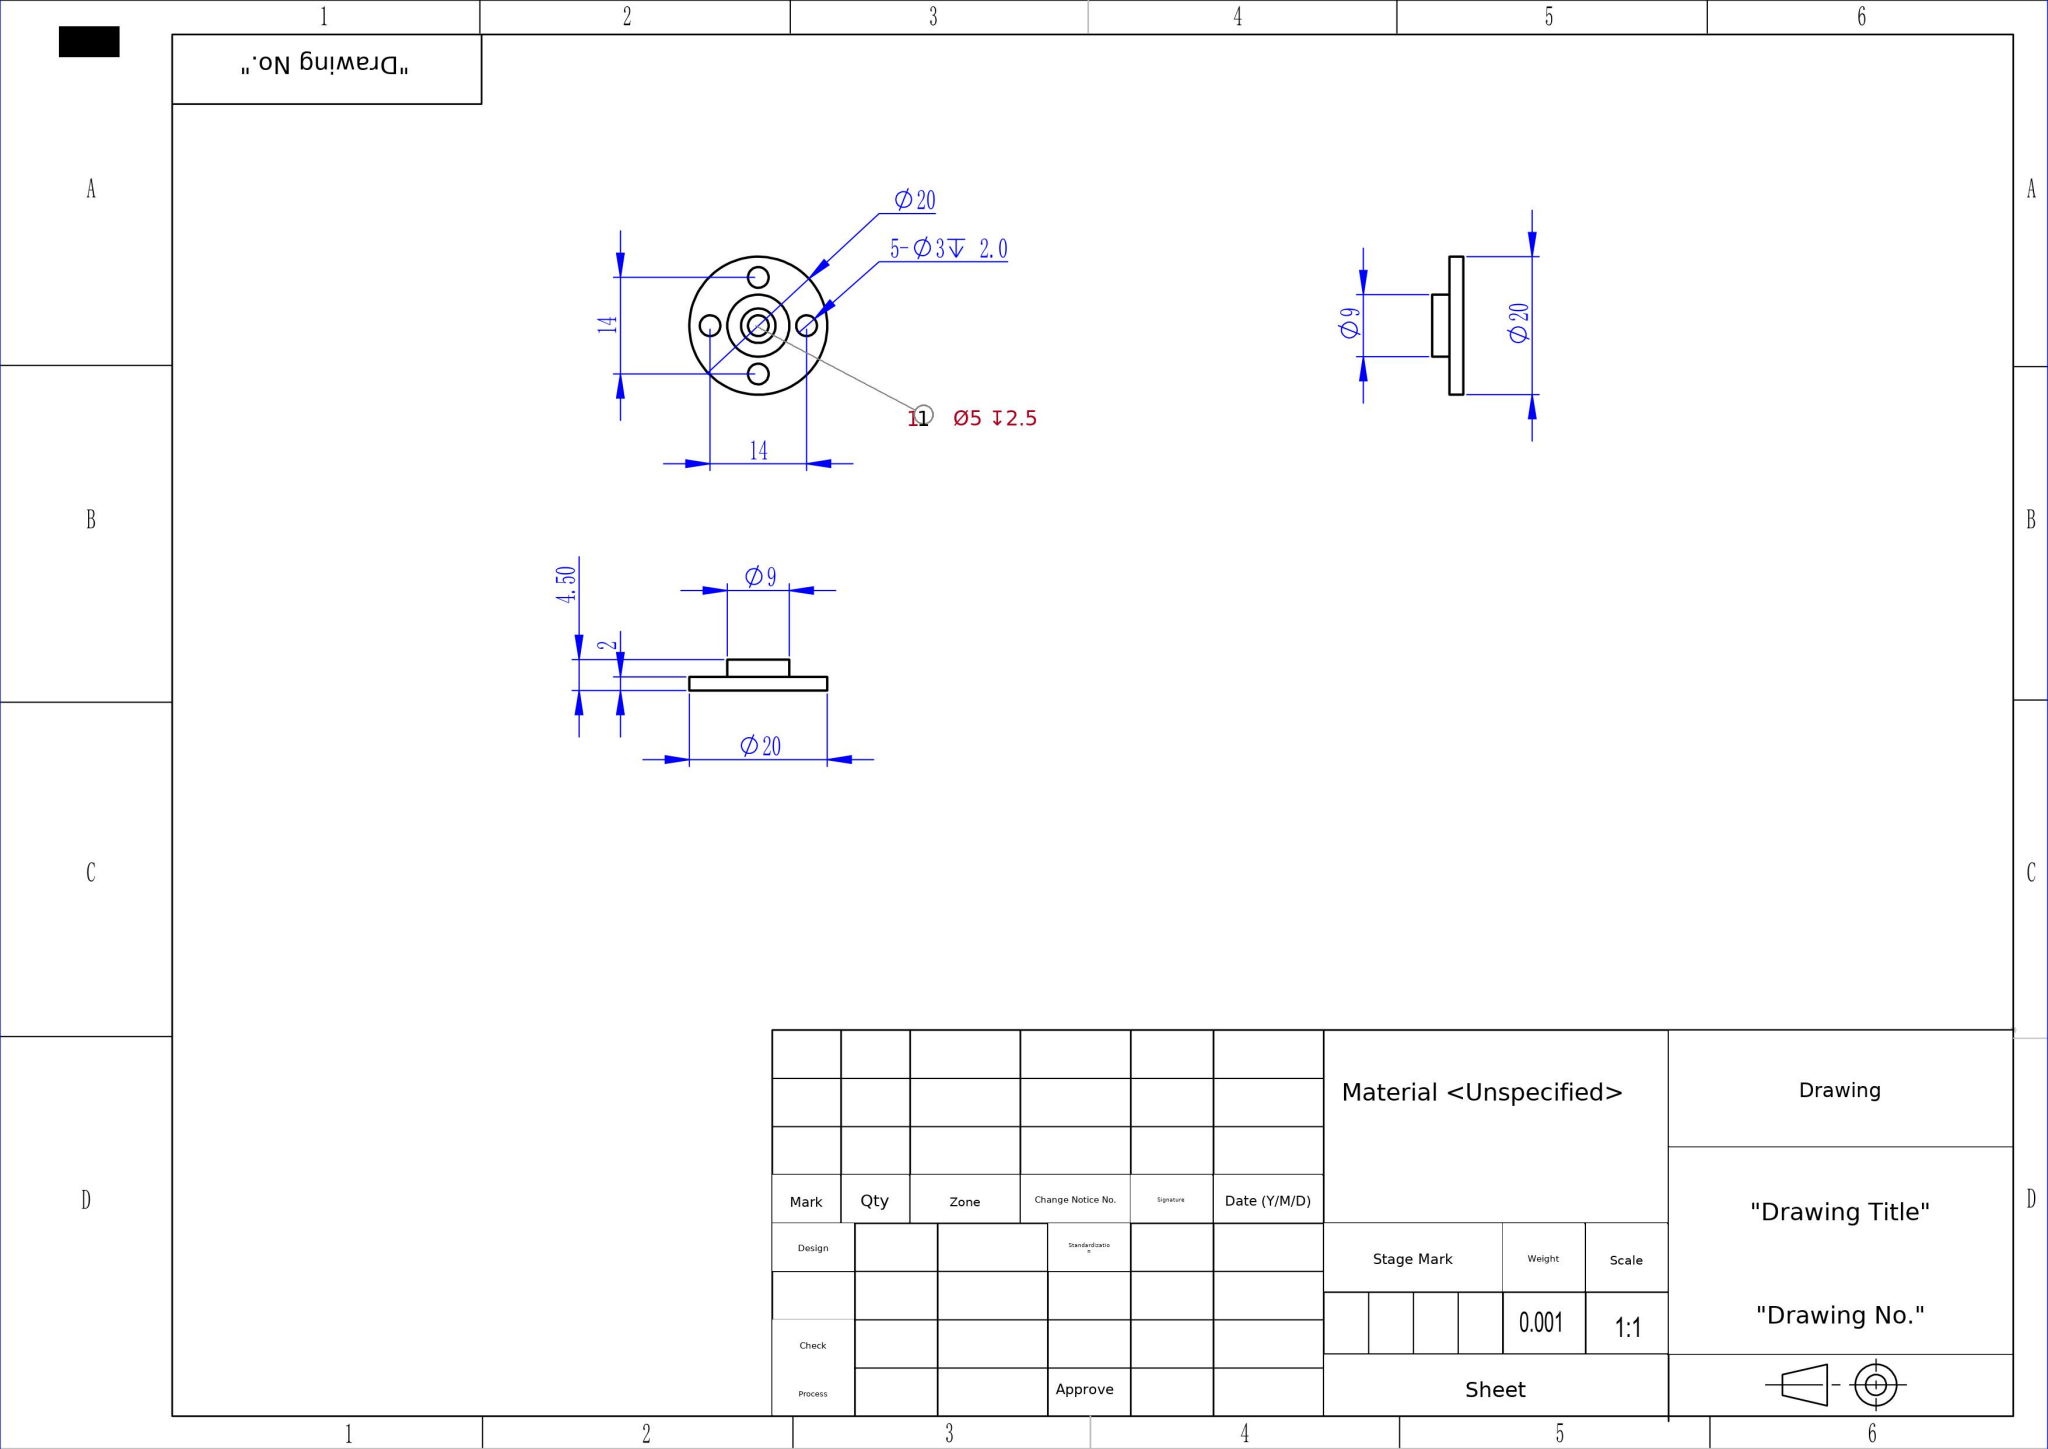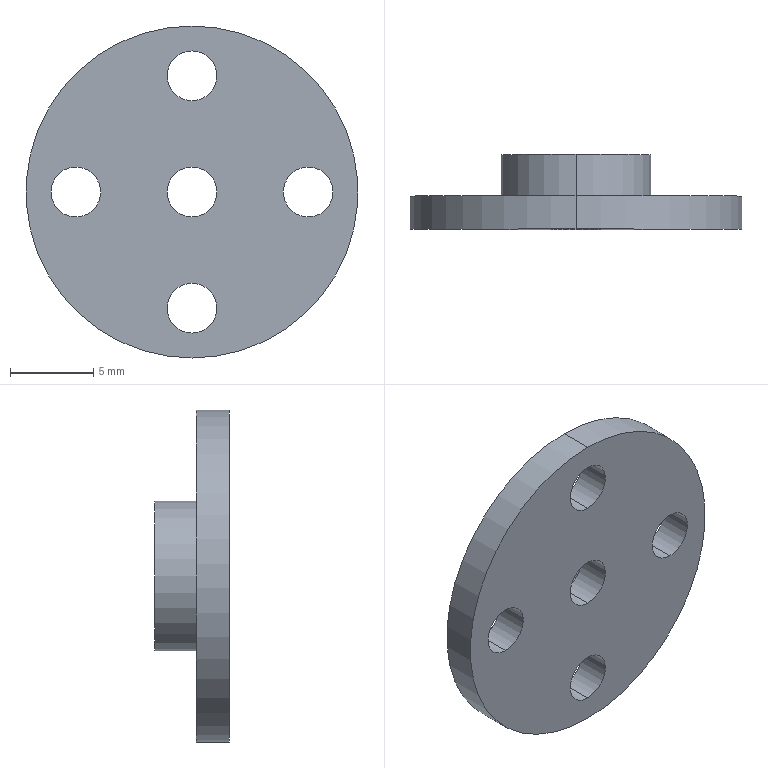Part | SolidWorks | mm | 1 solid | 20 faces | box 20 x 4.5 x 20 mm | volume 668 mm3 | cylinder 16 | plane 4 | commonest cylinder face diameters 3 x10 5 x2 9 x2 20 x2
build123d program:
from build123d import *

# Parameters (mm, degrees)
SKETCH1_R           = 10
BOSS_EXTRUDE1_DEPTH = 2
SKETCH2_R           = 1.5
CUT_EXTRUDE1_DEPTH  = 2
SKETCH3_R           = 4.5
SKETCH3_R_2         = 2.5
BOSS_EXTRUDE2_DEPTH = 2.5


with BuildPart() as part:
    # Sketch1 → Boss-Extrude1 (new body)
    with BuildSketch(Plane(origin=(0, 0, 0), x_dir=(1, 0, 0), z_dir=(0, 1, 0))):
        with Locations(Location((0, 0, 0), (0, 0, 270))):
            Circle(SKETCH1_R)
    extrude(amount=BOSS_EXTRUDE1_DEPTH)

    # Sketch2 → Cut-Extrude1 (cut)
    with BuildSketch(Plane(origin=(0, 2, 0), x_dir=(1, 0, 0), z_dir=(0, 1, 0))):
        with Locations(Location((0, 0, 0), (0, 0, 270))):
            Circle(SKETCH2_R)
        with Locations(Location((0, 7, 0), (0, 0, 270))):
            Circle(SKETCH2_R)
        with Locations(Location((7, 0, 0), (0, 0, 270))):
            Circle(SKETCH2_R)
        with Locations(Location((0, -7, 0), (0, 0, 270))):
            Circle(SKETCH2_R)
        with Locations(Location((-7, 0, 0), (0, 0, 270))):
            Circle(SKETCH2_R)
    extrude(amount=-CUT_EXTRUDE1_DEPTH, mode=Mode.SUBTRACT)

    # Sketch3 → Boss-Extrude2 (add)
    with BuildSketch(Plane(origin=(0, 2, 0), x_dir=(1, 0, 0), z_dir=(0, 1, 0))):
        with Locations(Location((0, 0, 0), (0, 0, 270))):
            Circle(SKETCH3_R)
        with Locations(Location((0, 0, 0), (0, 0, 270))):
            Circle(SKETCH3_R_2, mode=Mode.SUBTRACT)
    extrude(amount=BOSS_EXTRUDE2_DEPTH)


solid = part.part
STEP:
#1=CARTESIAN_POINT('',(0.,4.5,-2.5));
#2=VERTEX_POINT('',#1);
#3=CARTESIAN_POINT('',(0.,4.5,2.5));
#4=VERTEX_POINT('',#3);
#5=CARTESIAN_POINT('',(0.,4.5,0.));
#6=DIRECTION('',(0.,1.,0.));
#7=DIRECTION('',(0.,0.,1.));
#8=AXIS2_PLACEMENT_3D('',#5,#6,#7);
#9=CIRCLE('',#8,2.5);
#10=EDGE_CURVE('',#2,#4,#9,.T.);
#11=ORIENTED_EDGE('',*,*,#10,.T.);
#12=CARTESIAN_POINT('',(0.,2.,2.5));
#13=VERTEX_POINT('',#12);
#14=CARTESIAN_POINT('',(0.,4.5,2.5));
#15=DIRECTION('',(0.,-1.,0.));
#16=VECTOR('',#15,1000.);
#17=LINE('',#14,#16);
#18=EDGE_CURVE('',#4,#13,#17,.T.);
#19=ORIENTED_EDGE('',*,*,#18,.T.);
#20=CARTESIAN_POINT('',(0.,2.,-2.5));
#21=VERTEX_POINT('',#20);
#22=CARTESIAN_POINT('',(0.,2.,0.));
#23=DIRECTION('',(0.,-1.,0.));
#24=DIRECTION('',(0.,0.,1.));
#25=AXIS2_PLACEMENT_3D('',#22,#23,#24);
#26=CIRCLE('',#25,2.5);
#27=EDGE_CURVE('',#13,#21,#26,.T.);
#28=ORIENTED_EDGE('',*,*,#27,.T.);
#29=CARTESIAN_POINT('',(0.,4.5,-2.5));
#30=DIRECTION('',(0.,-1.,0.));
#31=VECTOR('',#30,1000.);
#32=LINE('',#29,#31);
#33=EDGE_CURVE('',#2,#21,#32,.T.);
#34=ORIENTED_EDGE('',*,*,#33,.F.);
#35=EDGE_LOOP('',(#11,#19,#28,#34));
#36=FACE_OUTER_BOUND('',#35,.T.);
#37=CARTESIAN_POINT('',(0.,4.5,0.));
#38=DIRECTION('',(0.,-1.,0.));
#39=DIRECTION('',(0.,0.,-1.));
#40=AXIS2_PLACEMENT_3D('',#37,#38,#39);
#41=CYLINDRICAL_SURFACE('',#40,2.5);
#42=ADVANCED_FACE('',(#36),#41,.F.);
#43=CARTESIAN_POINT('',(0.,4.5,4.5));
#44=VERTEX_POINT('',#43);
#45=CARTESIAN_POINT('',(0.,4.5,-4.5));
#46=VERTEX_POINT('',#45);
#47=CARTESIAN_POINT('',(0.,4.5,0.));
#48=DIRECTION('',(0.,1.,0.));
#49=DIRECTION('',(0.,0.,1.));
#50=AXIS2_PLACEMENT_3D('',#47,#48,#49);
#51=CIRCLE('',#50,4.5);
#52=EDGE_CURVE('',#44,#46,#51,.T.);
#53=ORIENTED_EDGE('',*,*,#52,.F.);
#54=CARTESIAN_POINT('',(0.,2.,4.5));
#55=VERTEX_POINT('',#54);
#56=CARTESIAN_POINT('',(0.,4.5,4.5));
#57=DIRECTION('',(0.,-1.,0.));
#58=VECTOR('',#57,1000.);
#59=LINE('',#56,#58);
#60=EDGE_CURVE('',#44,#55,#59,.T.);
#61=ORIENTED_EDGE('',*,*,#60,.T.);
#62=CARTESIAN_POINT('',(0.,2.,-4.5));
#63=VERTEX_POINT('',#62);
#64=CARTESIAN_POINT('',(0.,2.,0.));
#65=DIRECTION('',(0.,1.,0.));
#66=DIRECTION('',(0.,0.,1.));
#67=AXIS2_PLACEMENT_3D('',#64,#65,#66);
#68=CIRCLE('',#67,4.5);
#69=EDGE_CURVE('',#55,#63,#68,.T.);
#70=ORIENTED_EDGE('',*,*,#69,.T.);
#71=CARTESIAN_POINT('',(0.,4.5,-4.5));
#72=DIRECTION('',(0.,-1.,0.));
#73=VECTOR('',#72,1000.);
#74=LINE('',#71,#73);
#75=EDGE_CURVE('',#46,#63,#74,.T.);
#76=ORIENTED_EDGE('',*,*,#75,.F.);
#77=EDGE_LOOP('',(#53,#61,#70,#76));
#78=FACE_OUTER_BOUND('',#77,.T.);
#79=CARTESIAN_POINT('',(0.,4.5,0.));
#80=DIRECTION('',(0.,-1.,0.));
#81=DIRECTION('',(0.,0.,-1.));
#82=AXIS2_PLACEMENT_3D('',#79,#80,#81);
#83=CYLINDRICAL_SURFACE('',#82,4.5);
#84=ADVANCED_FACE('',(#78),#83,.T.);
#85=CARTESIAN_POINT('',(-7.,0.,-1.5));
#86=VERTEX_POINT('',#85);
#87=CARTESIAN_POINT('',(-7.,0.,1.5));
#88=VERTEX_POINT('',#87);
#89=CARTESIAN_POINT('',(-7.,0.,0.));
#90=DIRECTION('',(0.,1.,0.));
#91=DIRECTION('',(0.,0.,1.));
#92=AXIS2_PLACEMENT_3D('',#89,#90,#91);
#93=CIRCLE('',#92,1.5);
#94=EDGE_CURVE('',#86,#88,#93,.T.);
#95=ORIENTED_EDGE('',*,*,#94,.F.);
#96=CARTESIAN_POINT('',(-7.,2.,-1.5));
#97=VERTEX_POINT('',#96);
#98=CARTESIAN_POINT('',(-7.,0.,-1.5));
#99=DIRECTION('',(0.,1.,0.));
#100=VECTOR('',#99,1000.);
#101=LINE('',#98,#100);
#102=EDGE_CURVE('',#86,#97,#101,.T.);
#103=ORIENTED_EDGE('',*,*,#102,.T.);
#104=CARTESIAN_POINT('',(-7.,2.,1.5));
#105=VERTEX_POINT('',#104);
#106=CARTESIAN_POINT('',(-7.,2.,0.));
#107=DIRECTION('',(0.,1.,0.));
#108=DIRECTION('',(0.,0.,1.));
#109=AXIS2_PLACEMENT_3D('',#106,#107,#108);
#110=CIRCLE('',#109,1.5);
#111=EDGE_CURVE('',#97,#105,#110,.T.);
#112=ORIENTED_EDGE('',*,*,#111,.T.);
#113=CARTESIAN_POINT('',(-7.,0.,1.5));
#114=DIRECTION('',(0.,1.,0.));
#115=VECTOR('',#114,1000.);
#116=LINE('',#113,#115);
#117=EDGE_CURVE('',#88,#105,#116,.T.);
#118=ORIENTED_EDGE('',*,*,#117,.F.);
#119=EDGE_LOOP('',(#95,#103,#112,#118));
#120=FACE_OUTER_BOUND('',#119,.T.);
#121=CARTESIAN_POINT('',(-7.,0.,0.));
#122=DIRECTION('',(0.,1.,0.));
#123=DIRECTION('',(0.,0.,1.));
#124=AXIS2_PLACEMENT_3D('',#121,#122,#123);
#125=CYLINDRICAL_SURFACE('',#124,1.5);
#126=ADVANCED_FACE('',(#120),#125,.F.);
#127=CARTESIAN_POINT('',(0.,0.,5.5));
#128=VERTEX_POINT('',#127);
#129=CARTESIAN_POINT('',(0.,0.,8.5));
#130=VERTEX_POINT('',#129);
#131=CARTESIAN_POINT('',(0.,0.,7.));
#132=DIRECTION('',(0.,1.,0.));
#133=DIRECTION('',(0.,0.,1.));
#134=AXIS2_PLACEMENT_3D('',#131,#132,#133);
#135=CIRCLE('',#134,1.5);
#136=EDGE_CURVE('',#128,#130,#135,.T.);
#137=ORIENTED_EDGE('',*,*,#136,.F.);
#138=CARTESIAN_POINT('',(0.,2.,5.5));
#139=VERTEX_POINT('',#138);
#140=CARTESIAN_POINT('',(0.,0.,5.5));
#141=DIRECTION('',(0.,1.,0.));
#142=VECTOR('',#141,1000.);
#143=LINE('',#140,#142);
#144=EDGE_CURVE('',#128,#139,#143,.T.);
#145=ORIENTED_EDGE('',*,*,#144,.T.);
#146=CARTESIAN_POINT('',(0.,2.,8.5));
#147=VERTEX_POINT('',#146);
#148=CARTESIAN_POINT('',(0.,2.,7.));
#149=DIRECTION('',(0.,1.,0.));
#150=DIRECTION('',(0.,0.,1.));
#151=AXIS2_PLACEMENT_3D('',#148,#149,#150);
#152=CIRCLE('',#151,1.5);
#153=EDGE_CURVE('',#139,#147,#152,.T.);
#154=ORIENTED_EDGE('',*,*,#153,.T.);
#155=CARTESIAN_POINT('',(0.,0.,8.5));
#156=DIRECTION('',(0.,1.,0.));
#157=VECTOR('',#156,1000.);
#158=LINE('',#155,#157);
#159=EDGE_CURVE('',#130,#147,#158,.T.);
#160=ORIENTED_EDGE('',*,*,#159,.F.);
#161=EDGE_LOOP('',(#137,#145,#154,#160));
#162=FACE_OUTER_BOUND('',#161,.T.);
#163=CARTESIAN_POINT('',(0.,0.,7.));
#164=DIRECTION('',(0.,1.,0.));
#165=DIRECTION('',(0.,0.,1.));
#166=AXIS2_PLACEMENT_3D('',#163,#164,#165);
#167=CYLINDRICAL_SURFACE('',#166,1.5);
#168=ADVANCED_FACE('',(#162),#167,.F.);
#169=CARTESIAN_POINT('',(7.,0.,-1.5));
#170=VERTEX_POINT('',#169);
#171=CARTESIAN_POINT('',(7.,0.,1.5));
#172=VERTEX_POINT('',#171);
#173=CARTESIAN_POINT('',(7.,0.,-0.));
#174=DIRECTION('',(0.,1.,0.));
#175=DIRECTION('',(0.,0.,1.));
#176=AXIS2_PLACEMENT_3D('',#173,#174,#175);
#177=CIRCLE('',#176,1.5);
#178=EDGE_CURVE('',#170,#172,#177,.T.);
#179=ORIENTED_EDGE('',*,*,#178,.F.);
#180=CARTESIAN_POINT('',(7.,2.,-1.5));
#181=VERTEX_POINT('',#180);
#182=CARTESIAN_POINT('',(7.,0.,-1.5));
#183=DIRECTION('',(0.,1.,0.));
#184=VECTOR('',#183,1000.);
#185=LINE('',#182,#184);
#186=EDGE_CURVE('',#170,#181,#185,.T.);
#187=ORIENTED_EDGE('',*,*,#186,.T.);
#188=CARTESIAN_POINT('',(7.,2.,1.5));
#189=VERTEX_POINT('',#188);
#190=CARTESIAN_POINT('',(7.,2.,-0.));
#191=DIRECTION('',(0.,1.,0.));
#192=DIRECTION('',(0.,0.,1.));
#193=AXIS2_PLACEMENT_3D('',#190,#191,#192);
#194=CIRCLE('',#193,1.5);
#195=EDGE_CURVE('',#181,#189,#194,.T.);
#196=ORIENTED_EDGE('',*,*,#195,.T.);
#197=CARTESIAN_POINT('',(7.,0.,1.5));
#198=DIRECTION('',(0.,1.,0.));
#199=VECTOR('',#198,1000.);
#200=LINE('',#197,#199);
#201=EDGE_CURVE('',#172,#189,#200,.T.);
#202=ORIENTED_EDGE('',*,*,#201,.F.);
#203=EDGE_LOOP('',(#179,#187,#196,#202));
#204=FACE_OUTER_BOUND('',#203,.T.);
#205=CARTESIAN_POINT('',(7.,0.,-0.));
#206=DIRECTION('',(0.,1.,0.));
#207=DIRECTION('',(0.,0.,1.));
#208=AXIS2_PLACEMENT_3D('',#205,#206,#207);
#209=CYLINDRICAL_SURFACE('',#208,1.5);
#210=ADVANCED_FACE('',(#204),#209,.F.);
#211=CARTESIAN_POINT('',(0.,0.,-8.5));
#212=VERTEX_POINT('',#211);
#213=CARTESIAN_POINT('',(0.,0.,-5.5));
#214=VERTEX_POINT('',#213);
#215=CARTESIAN_POINT('',(0.,0.,-7.));
#216=DIRECTION('',(0.,1.,0.));
#217=DIRECTION('',(0.,0.,1.));
#218=AXIS2_PLACEMENT_3D('',#215,#216,#217);
#219=CIRCLE('',#218,1.5);
#220=EDGE_CURVE('',#212,#214,#219,.T.);
#221=ORIENTED_EDGE('',*,*,#220,.F.);
#222=CARTESIAN_POINT('',(0.,2.,-8.5));
#223=VERTEX_POINT('',#222);
#224=CARTESIAN_POINT('',(0.,0.,-8.5));
#225=DIRECTION('',(0.,1.,0.));
#226=VECTOR('',#225,1000.);
#227=LINE('',#224,#226);
#228=EDGE_CURVE('',#212,#223,#227,.T.);
#229=ORIENTED_EDGE('',*,*,#228,.T.);
#230=CARTESIAN_POINT('',(0.,2.,-5.5));
#231=VERTEX_POINT('',#230);
#232=CARTESIAN_POINT('',(0.,2.,-7.));
#233=DIRECTION('',(0.,1.,0.));
#234=DIRECTION('',(0.,0.,1.));
#235=AXIS2_PLACEMENT_3D('',#232,#233,#234);
#236=CIRCLE('',#235,1.5);
#237=EDGE_CURVE('',#223,#231,#236,.T.);
#238=ORIENTED_EDGE('',*,*,#237,.T.);
#239=CARTESIAN_POINT('',(0.,0.,-5.5));
#240=DIRECTION('',(0.,1.,0.));
#241=VECTOR('',#240,1000.);
#242=LINE('',#239,#241);
#243=EDGE_CURVE('',#214,#231,#242,.T.);
#244=ORIENTED_EDGE('',*,*,#243,.F.);
#245=EDGE_LOOP('',(#221,#229,#238,#244));
#246=FACE_OUTER_BOUND('',#245,.T.);
#247=CARTESIAN_POINT('',(0.,0.,-7.));
#248=DIRECTION('',(0.,1.,0.));
#249=DIRECTION('',(0.,0.,1.));
#250=AXIS2_PLACEMENT_3D('',#247,#248,#249);
#251=CYLINDRICAL_SURFACE('',#250,1.5);
#252=ADVANCED_FACE('',(#246),#251,.F.);
#253=CARTESIAN_POINT('',(0.,0.,-1.5));
#254=VERTEX_POINT('',#253);
#255=CARTESIAN_POINT('',(0.,0.,1.5));
#256=VERTEX_POINT('',#255);
#257=CARTESIAN_POINT('',(0.,0.,0.));
#258=DIRECTION('',(0.,1.,0.));
#259=DIRECTION('',(0.,0.,1.));
#260=AXIS2_PLACEMENT_3D('',#257,#258,#259);
#261=CIRCLE('',#260,1.5);
#262=EDGE_CURVE('',#254,#256,#261,.T.);
#263=ORIENTED_EDGE('',*,*,#262,.F.);
#264=CARTESIAN_POINT('',(0.,2.,-1.5));
#265=VERTEX_POINT('',#264);
#266=CARTESIAN_POINT('',(0.,0.,-1.5));
#267=DIRECTION('',(0.,1.,0.));
#268=VECTOR('',#267,1000.);
#269=LINE('',#266,#268);
#270=EDGE_CURVE('',#254,#265,#269,.T.);
#271=ORIENTED_EDGE('',*,*,#270,.T.);
#272=CARTESIAN_POINT('',(0.,2.,1.5));
#273=VERTEX_POINT('',#272);
#274=CARTESIAN_POINT('',(0.,2.,0.));
#275=DIRECTION('',(0.,1.,0.));
#276=DIRECTION('',(0.,0.,1.));
#277=AXIS2_PLACEMENT_3D('',#274,#275,#276);
#278=CIRCLE('',#277,1.5);
#279=EDGE_CURVE('',#265,#273,#278,.T.);
#280=ORIENTED_EDGE('',*,*,#279,.T.);
#281=CARTESIAN_POINT('',(0.,0.,1.5));
#282=DIRECTION('',(0.,1.,0.));
#283=VECTOR('',#282,1000.);
#284=LINE('',#281,#283);
#285=EDGE_CURVE('',#256,#273,#284,.T.);
#286=ORIENTED_EDGE('',*,*,#285,.F.);
#287=EDGE_LOOP('',(#263,#271,#280,#286));
#288=FACE_OUTER_BOUND('',#287,.T.);
#289=CARTESIAN_POINT('',(0.,0.,0.));
#290=DIRECTION('',(0.,1.,0.));
#291=DIRECTION('',(0.,0.,1.));
#292=AXIS2_PLACEMENT_3D('',#289,#290,#291);
#293=CYLINDRICAL_SURFACE('',#292,1.5);
#294=ADVANCED_FACE('',(#288),#293,.F.);
#295=CARTESIAN_POINT('',(0.,2.,10.));
#296=VERTEX_POINT('',#295);
#297=CARTESIAN_POINT('',(0.,2.,-10.));
#298=VERTEX_POINT('',#297);
#299=CARTESIAN_POINT('',(0.,2.,0.));
#300=DIRECTION('',(0.,1.,0.));
#301=DIRECTION('',(0.,0.,1.));
#302=AXIS2_PLACEMENT_3D('',#299,#300,#301);
#303=CIRCLE('',#302,10.);
#304=EDGE_CURVE('',#296,#298,#303,.T.);
#305=ORIENTED_EDGE('',*,*,#304,.F.);
#306=CARTESIAN_POINT('',(0.,0.,10.));
#307=VERTEX_POINT('',#306);
#308=CARTESIAN_POINT('',(0.,2.,10.));
#309=DIRECTION('',(0.,-1.,0.));
#310=VECTOR('',#309,1000.);
#311=LINE('',#308,#310);
#312=EDGE_CURVE('',#296,#307,#311,.T.);
#313=ORIENTED_EDGE('',*,*,#312,.T.);
#314=CARTESIAN_POINT('',(0.,0.,-10.));
#315=VERTEX_POINT('',#314);
#316=CARTESIAN_POINT('',(0.,0.,0.));
#317=DIRECTION('',(0.,1.,0.));
#318=DIRECTION('',(0.,0.,1.));
#319=AXIS2_PLACEMENT_3D('',#316,#317,#318);
#320=CIRCLE('',#319,10.);
#321=EDGE_CURVE('',#307,#315,#320,.T.);
#322=ORIENTED_EDGE('',*,*,#321,.T.);
#323=CARTESIAN_POINT('',(0.,2.,-10.));
#324=DIRECTION('',(0.,-1.,0.));
#325=VECTOR('',#324,1000.);
#326=LINE('',#323,#325);
#327=EDGE_CURVE('',#298,#315,#326,.T.);
#328=ORIENTED_EDGE('',*,*,#327,.F.);
#329=EDGE_LOOP('',(#305,#313,#322,#328));
#330=FACE_OUTER_BOUND('',#329,.T.);
#331=CARTESIAN_POINT('',(0.,2.,0.));
#332=DIRECTION('',(0.,-1.,0.));
#333=DIRECTION('',(0.,0.,-1.));
#334=AXIS2_PLACEMENT_3D('',#331,#332,#333);
#335=CYLINDRICAL_SURFACE('',#334,10.);
#336=ADVANCED_FACE('',(#330),#335,.T.);
#337=CARTESIAN_POINT('',(0.,2.,0.));
#338=DIRECTION('',(0.,1.,0.));
#339=DIRECTION('',(0.,0.,1.));
#340=AXIS2_PLACEMENT_3D('',#337,#338,#339);
#341=CIRCLE('',#340,1.5);
#342=EDGE_CURVE('',#273,#265,#341,.T.);
#343=ORIENTED_EDGE('',*,*,#342,.F.);
#344=ORIENTED_EDGE('',*,*,#279,.F.);
#345=EDGE_LOOP('',(#343,#344));
#346=FACE_BOUND('',#345,.T.);
#347=CARTESIAN_POINT('',(0.,2.,0.));
#348=DIRECTION('',(0.,-1.,0.));
#349=DIRECTION('',(0.,0.,1.));
#350=AXIS2_PLACEMENT_3D('',#347,#348,#349);
#351=CIRCLE('',#350,2.5);
#352=EDGE_CURVE('',#21,#13,#351,.T.);
#353=ORIENTED_EDGE('',*,*,#352,.F.);
#354=ORIENTED_EDGE('',*,*,#27,.F.);
#355=EDGE_LOOP('',(#353,#354));
#356=FACE_OUTER_BOUND('',#355,.T.);
#357=CARTESIAN_POINT('',(0.,2.,0.));
#358=DIRECTION('',(0.,1.,0.));
#359=DIRECTION('',(0.,0.,1.));
#360=AXIS2_PLACEMENT_3D('',#357,#358,#359);
#361=PLANE('',#360);
#362=ADVANCED_FACE('',(#346,#356),#361,.T.);
#363=ORIENTED_EDGE('',*,*,#312,.F.);
#364=CARTESIAN_POINT('',(0.,2.,0.));
#365=DIRECTION('',(0.,1.,0.));
#366=DIRECTION('',(0.,0.,1.));
#367=AXIS2_PLACEMENT_3D('',#364,#365,#366);
#368=CIRCLE('',#367,10.);
#369=EDGE_CURVE('',#298,#296,#368,.T.);
#370=ORIENTED_EDGE('',*,*,#369,.F.);
#371=ORIENTED_EDGE('',*,*,#327,.T.);
#372=CARTESIAN_POINT('',(0.,0.,0.));
#373=DIRECTION('',(0.,1.,0.));
#374=DIRECTION('',(0.,0.,1.));
#375=AXIS2_PLACEMENT_3D('',#372,#373,#374);
#376=CIRCLE('',#375,10.);
#377=EDGE_CURVE('',#315,#307,#376,.T.);
#378=ORIENTED_EDGE('',*,*,#377,.T.);
#379=EDGE_LOOP('',(#363,#370,#371,#378));
#380=FACE_OUTER_BOUND('',#379,.T.);
#381=CARTESIAN_POINT('',(0.,2.,0.));
#382=DIRECTION('',(0.,-1.,0.));
#383=DIRECTION('',(0.,0.,-1.));
#384=AXIS2_PLACEMENT_3D('',#381,#382,#383);
#385=CYLINDRICAL_SURFACE('',#384,10.);
#386=ADVANCED_FACE('',(#380),#385,.T.);
#387=CARTESIAN_POINT('',(0.,2.,0.));
#388=DIRECTION('',(0.,1.,0.));
#389=DIRECTION('',(0.,0.,1.));
#390=AXIS2_PLACEMENT_3D('',#387,#388,#389);
#391=CIRCLE('',#390,4.5);
#392=EDGE_CURVE('',#63,#55,#391,.T.);
#393=ORIENTED_EDGE('',*,*,#392,.F.);
#394=ORIENTED_EDGE('',*,*,#69,.F.);
#395=EDGE_LOOP('',(#393,#394));
#396=FACE_BOUND('',#395,.T.);
#397=CARTESIAN_POINT('',(-7.,2.,0.));
#398=DIRECTION('',(0.,1.,0.));
#399=DIRECTION('',(0.,0.,1.));
#400=AXIS2_PLACEMENT_3D('',#397,#398,#399);
#401=CIRCLE('',#400,1.5);
#402=EDGE_CURVE('',#105,#97,#401,.T.);
#403=ORIENTED_EDGE('',*,*,#402,.F.);
#404=ORIENTED_EDGE('',*,*,#111,.F.);
#405=EDGE_LOOP('',(#403,#404));
#406=FACE_BOUND('',#405,.T.);
#407=CARTESIAN_POINT('',(0.,2.,7.));
#408=DIRECTION('',(0.,1.,0.));
#409=DIRECTION('',(0.,0.,1.));
#410=AXIS2_PLACEMENT_3D('',#407,#408,#409);
#411=CIRCLE('',#410,1.5);
#412=EDGE_CURVE('',#147,#139,#411,.T.);
#413=ORIENTED_EDGE('',*,*,#412,.F.);
#414=ORIENTED_EDGE('',*,*,#153,.F.);
#415=EDGE_LOOP('',(#413,#414));
#416=FACE_BOUND('',#415,.T.);
#417=CARTESIAN_POINT('',(7.,2.,-0.));
#418=DIRECTION('',(0.,1.,0.));
#419=DIRECTION('',(0.,0.,1.));
#420=AXIS2_PLACEMENT_3D('',#417,#418,#419);
#421=CIRCLE('',#420,1.5);
#422=EDGE_CURVE('',#189,#181,#421,.T.);
#423=ORIENTED_EDGE('',*,*,#422,.F.);
#424=ORIENTED_EDGE('',*,*,#195,.F.);
#425=EDGE_LOOP('',(#423,#424));
#426=FACE_BOUND('',#425,.T.);
#427=CARTESIAN_POINT('',(0.,2.,-7.));
#428=DIRECTION('',(0.,1.,0.));
#429=DIRECTION('',(0.,0.,1.));
#430=AXIS2_PLACEMENT_3D('',#427,#428,#429);
#431=CIRCLE('',#430,1.5);
#432=EDGE_CURVE('',#231,#223,#431,.T.);
#433=ORIENTED_EDGE('',*,*,#432,.F.);
#434=ORIENTED_EDGE('',*,*,#237,.F.);
#435=EDGE_LOOP('',(#433,#434));
#436=FACE_BOUND('',#435,.T.);
#437=ORIENTED_EDGE('',*,*,#369,.T.);
#438=ORIENTED_EDGE('',*,*,#304,.T.);
#439=EDGE_LOOP('',(#437,#438));
#440=FACE_OUTER_BOUND('',#439,.T.);
#441=CARTESIAN_POINT('',(0.,2.,0.));
#442=DIRECTION('',(0.,1.,0.));
#443=DIRECTION('',(0.,0.,1.));
#444=AXIS2_PLACEMENT_3D('',#441,#442,#443);
#445=PLANE('',#444);
#446=ADVANCED_FACE('',(#396,#406,#416,#426,#436,#440),#445,.T.);
#447=CARTESIAN_POINT('',(-7.,0.,0.));
#448=DIRECTION('',(0.,1.,0.));
#449=DIRECTION('',(0.,0.,1.));
#450=AXIS2_PLACEMENT_3D('',#447,#448,#449);
#451=CIRCLE('',#450,1.5);
#452=EDGE_CURVE('',#88,#86,#451,.T.);
#453=ORIENTED_EDGE('',*,*,#452,.T.);
#454=ORIENTED_EDGE('',*,*,#94,.T.);
#455=EDGE_LOOP('',(#453,#454));
#456=FACE_BOUND('',#455,.T.);
#457=CARTESIAN_POINT('',(0.,0.,7.));
#458=DIRECTION('',(0.,1.,0.));
#459=DIRECTION('',(0.,0.,1.));
#460=AXIS2_PLACEMENT_3D('',#457,#458,#459);
#461=CIRCLE('',#460,1.5);
#462=EDGE_CURVE('',#130,#128,#461,.T.);
#463=ORIENTED_EDGE('',*,*,#462,.T.);
#464=ORIENTED_EDGE('',*,*,#136,.T.);
#465=EDGE_LOOP('',(#463,#464));
#466=FACE_BOUND('',#465,.T.);
#467=CARTESIAN_POINT('',(7.,0.,-0.));
#468=DIRECTION('',(0.,1.,0.));
#469=DIRECTION('',(0.,0.,1.));
#470=AXIS2_PLACEMENT_3D('',#467,#468,#469);
#471=CIRCLE('',#470,1.5);
#472=EDGE_CURVE('',#172,#170,#471,.T.);
#473=ORIENTED_EDGE('',*,*,#472,.T.);
#474=ORIENTED_EDGE('',*,*,#178,.T.);
#475=EDGE_LOOP('',(#473,#474));
#476=FACE_BOUND('',#475,.T.);
#477=CARTESIAN_POINT('',(0.,0.,-7.));
#478=DIRECTION('',(0.,1.,0.));
#479=DIRECTION('',(0.,0.,1.));
#480=AXIS2_PLACEMENT_3D('',#477,#478,#479);
#481=CIRCLE('',#480,1.5);
#482=EDGE_CURVE('',#214,#212,#481,.T.);
#483=ORIENTED_EDGE('',*,*,#482,.T.);
#484=ORIENTED_EDGE('',*,*,#220,.T.);
#485=EDGE_LOOP('',(#483,#484));
#486=FACE_BOUND('',#485,.T.);
#487=CARTESIAN_POINT('',(0.,0.,0.));
#488=DIRECTION('',(0.,1.,0.));
#489=DIRECTION('',(0.,0.,1.));
#490=AXIS2_PLACEMENT_3D('',#487,#488,#489);
#491=CIRCLE('',#490,1.5);
#492=EDGE_CURVE('',#256,#254,#491,.T.);
#493=ORIENTED_EDGE('',*,*,#492,.T.);
#494=ORIENTED_EDGE('',*,*,#262,.T.);
#495=EDGE_LOOP('',(#493,#494));
#496=FACE_BOUND('',#495,.T.);
#497=ORIENTED_EDGE('',*,*,#377,.F.);
#498=ORIENTED_EDGE('',*,*,#321,.F.);
#499=EDGE_LOOP('',(#497,#498));
#500=FACE_OUTER_BOUND('',#499,.T.);
#501=CARTESIAN_POINT('',(0.,0.,0.));
#502=DIRECTION('',(0.,1.,0.));
#503=DIRECTION('',(0.,0.,1.));
#504=AXIS2_PLACEMENT_3D('',#501,#502,#503);
#505=PLANE('',#504);
#506=ADVANCED_FACE('',(#456,#466,#476,#486,#496,#500),#505,.F.);
#507=ORIENTED_EDGE('',*,*,#270,.F.);
#508=ORIENTED_EDGE('',*,*,#492,.F.);
#509=ORIENTED_EDGE('',*,*,#285,.T.);
#510=ORIENTED_EDGE('',*,*,#342,.T.);
#511=EDGE_LOOP('',(#507,#508,#509,#510));
#512=FACE_OUTER_BOUND('',#511,.T.);
#513=CARTESIAN_POINT('',(0.,0.,0.));
#514=DIRECTION('',(0.,1.,0.));
#515=DIRECTION('',(0.,0.,1.));
#516=AXIS2_PLACEMENT_3D('',#513,#514,#515);
#517=CYLINDRICAL_SURFACE('',#516,1.5);
#518=ADVANCED_FACE('',(#512),#517,.F.);
#519=ORIENTED_EDGE('',*,*,#228,.F.);
#520=ORIENTED_EDGE('',*,*,#482,.F.);
#521=ORIENTED_EDGE('',*,*,#243,.T.);
#522=ORIENTED_EDGE('',*,*,#432,.T.);
#523=EDGE_LOOP('',(#519,#520,#521,#522));
#524=FACE_OUTER_BOUND('',#523,.T.);
#525=CARTESIAN_POINT('',(0.,0.,-7.));
#526=DIRECTION('',(0.,1.,0.));
#527=DIRECTION('',(0.,0.,1.));
#528=AXIS2_PLACEMENT_3D('',#525,#526,#527);
#529=CYLINDRICAL_SURFACE('',#528,1.5);
#530=ADVANCED_FACE('',(#524),#529,.F.);
#531=ORIENTED_EDGE('',*,*,#186,.F.);
#532=ORIENTED_EDGE('',*,*,#472,.F.);
#533=ORIENTED_EDGE('',*,*,#201,.T.);
#534=ORIENTED_EDGE('',*,*,#422,.T.);
#535=EDGE_LOOP('',(#531,#532,#533,#534));
#536=FACE_OUTER_BOUND('',#535,.T.);
#537=CARTESIAN_POINT('',(7.,0.,-0.));
#538=DIRECTION('',(0.,1.,0.));
#539=DIRECTION('',(0.,0.,1.));
#540=AXIS2_PLACEMENT_3D('',#537,#538,#539);
#541=CYLINDRICAL_SURFACE('',#540,1.5);
#542=ADVANCED_FACE('',(#536),#541,.F.);
#543=ORIENTED_EDGE('',*,*,#144,.F.);
#544=ORIENTED_EDGE('',*,*,#462,.F.);
#545=ORIENTED_EDGE('',*,*,#159,.T.);
#546=ORIENTED_EDGE('',*,*,#412,.T.);
#547=EDGE_LOOP('',(#543,#544,#545,#546));
#548=FACE_OUTER_BOUND('',#547,.T.);
#549=CARTESIAN_POINT('',(0.,0.,7.));
#550=DIRECTION('',(0.,1.,0.));
#551=DIRECTION('',(0.,0.,1.));
#552=AXIS2_PLACEMENT_3D('',#549,#550,#551);
#553=CYLINDRICAL_SURFACE('',#552,1.5);
#554=ADVANCED_FACE('',(#548),#553,.F.);
#555=ORIENTED_EDGE('',*,*,#102,.F.);
#556=ORIENTED_EDGE('',*,*,#452,.F.);
#557=ORIENTED_EDGE('',*,*,#117,.T.);
#558=ORIENTED_EDGE('',*,*,#402,.T.);
#559=EDGE_LOOP('',(#555,#556,#557,#558));
#560=FACE_OUTER_BOUND('',#559,.T.);
#561=CARTESIAN_POINT('',(-7.,0.,0.));
#562=DIRECTION('',(0.,1.,0.));
#563=DIRECTION('',(0.,0.,1.));
#564=AXIS2_PLACEMENT_3D('',#561,#562,#563);
#565=CYLINDRICAL_SURFACE('',#564,1.5);
#566=ADVANCED_FACE('',(#560),#565,.F.);
#567=CARTESIAN_POINT('',(0.,4.5,0.));
#568=DIRECTION('',(0.,1.,0.));
#569=DIRECTION('',(0.,0.,1.));
#570=AXIS2_PLACEMENT_3D('',#567,#568,#569);
#571=CIRCLE('',#570,4.5);
#572=EDGE_CURVE('',#46,#44,#571,.T.);
#573=ORIENTED_EDGE('',*,*,#572,.T.);
#574=ORIENTED_EDGE('',*,*,#52,.T.);
#575=EDGE_LOOP('',(#573,#574));
#576=FACE_OUTER_BOUND('',#575,.T.);
#577=ORIENTED_EDGE('',*,*,#10,.F.);
#578=CARTESIAN_POINT('',(0.,4.5,0.));
#579=DIRECTION('',(0.,1.,0.));
#580=DIRECTION('',(0.,0.,1.));
#581=AXIS2_PLACEMENT_3D('',#578,#579,#580);
#582=CIRCLE('',#581,2.5);
#583=EDGE_CURVE('',#4,#2,#582,.T.);
#584=ORIENTED_EDGE('',*,*,#583,.F.);
#585=EDGE_LOOP('',(#577,#584));
#586=FACE_BOUND('',#585,.T.);
#587=CARTESIAN_POINT('',(0.,4.5,0.));
#588=DIRECTION('',(0.,1.,0.));
#589=DIRECTION('',(0.,0.,1.));
#590=AXIS2_PLACEMENT_3D('',#587,#588,#589);
#591=PLANE('',#590);
#592=ADVANCED_FACE('',(#576,#586),#591,.T.);
#593=ORIENTED_EDGE('',*,*,#60,.F.);
#594=ORIENTED_EDGE('',*,*,#572,.F.);
#595=ORIENTED_EDGE('',*,*,#75,.T.);
#596=ORIENTED_EDGE('',*,*,#392,.T.);
#597=EDGE_LOOP('',(#593,#594,#595,#596));
#598=FACE_OUTER_BOUND('',#597,.T.);
#599=CARTESIAN_POINT('',(0.,4.5,0.));
#600=DIRECTION('',(0.,-1.,0.));
#601=DIRECTION('',(0.,0.,-1.));
#602=AXIS2_PLACEMENT_3D('',#599,#600,#601);
#603=CYLINDRICAL_SURFACE('',#602,4.5);
#604=ADVANCED_FACE('',(#598),#603,.T.);
#605=ORIENTED_EDGE('',*,*,#18,.F.);
#606=ORIENTED_EDGE('',*,*,#583,.T.);
#607=ORIENTED_EDGE('',*,*,#33,.T.);
#608=ORIENTED_EDGE('',*,*,#352,.T.);
#609=EDGE_LOOP('',(#605,#606,#607,#608));
#610=FACE_OUTER_BOUND('',#609,.T.);
#611=CARTESIAN_POINT('',(0.,4.5,0.));
#612=DIRECTION('',(0.,-1.,0.));
#613=DIRECTION('',(0.,0.,-1.));
#614=AXIS2_PLACEMENT_3D('',#611,#612,#613);
#615=CYLINDRICAL_SURFACE('',#614,2.5);
#616=ADVANCED_FACE('',(#610),#615,.F.);
#617=CLOSED_SHELL('',(#42,#84,#126,#168,#210,#252,#294,#336,#362,#386,#446,#506,#518,#530,#542,#554,#566,#592,#604,#616));
#618=MANIFOLD_SOLID_BREP('',#617);
#619=CARTESIAN_POINT('',(0.,0.,0.));
#620=DIRECTION('',(0.,0.,1.));
#621=DIRECTION('',(1.,0.,0.));
#622=AXIS2_PLACEMENT_3D('',#619,#620,#621);
#623=(LENGTH_UNIT()NAMED_UNIT(*)SI_UNIT(.MILLI.,.METRE.));
#624=UNCERTAINTY_MEASURE_WITH_UNIT(LENGTH_MEASURE(0.00001),#623,'','');
#625=(NAMED_UNIT(*)PLANE_ANGLE_UNIT()SI_UNIT($,.RADIAN.));
#626=(NAMED_UNIT(*)SI_UNIT($,.STERADIAN.)SOLID_ANGLE_UNIT());
#627=(GEOMETRIC_REPRESENTATION_CONTEXT(3)GLOBAL_UNCERTAINTY_ASSIGNED_CONTEXT((#624))GLOBAL_UNIT_ASSIGNED_CONTEXT((#623,#625,#626))REPRESENTATION_CONTEXT('',''));
#628=ADVANCED_BREP_SHAPE_REPRESENTATION('',(#618,#622),#627);